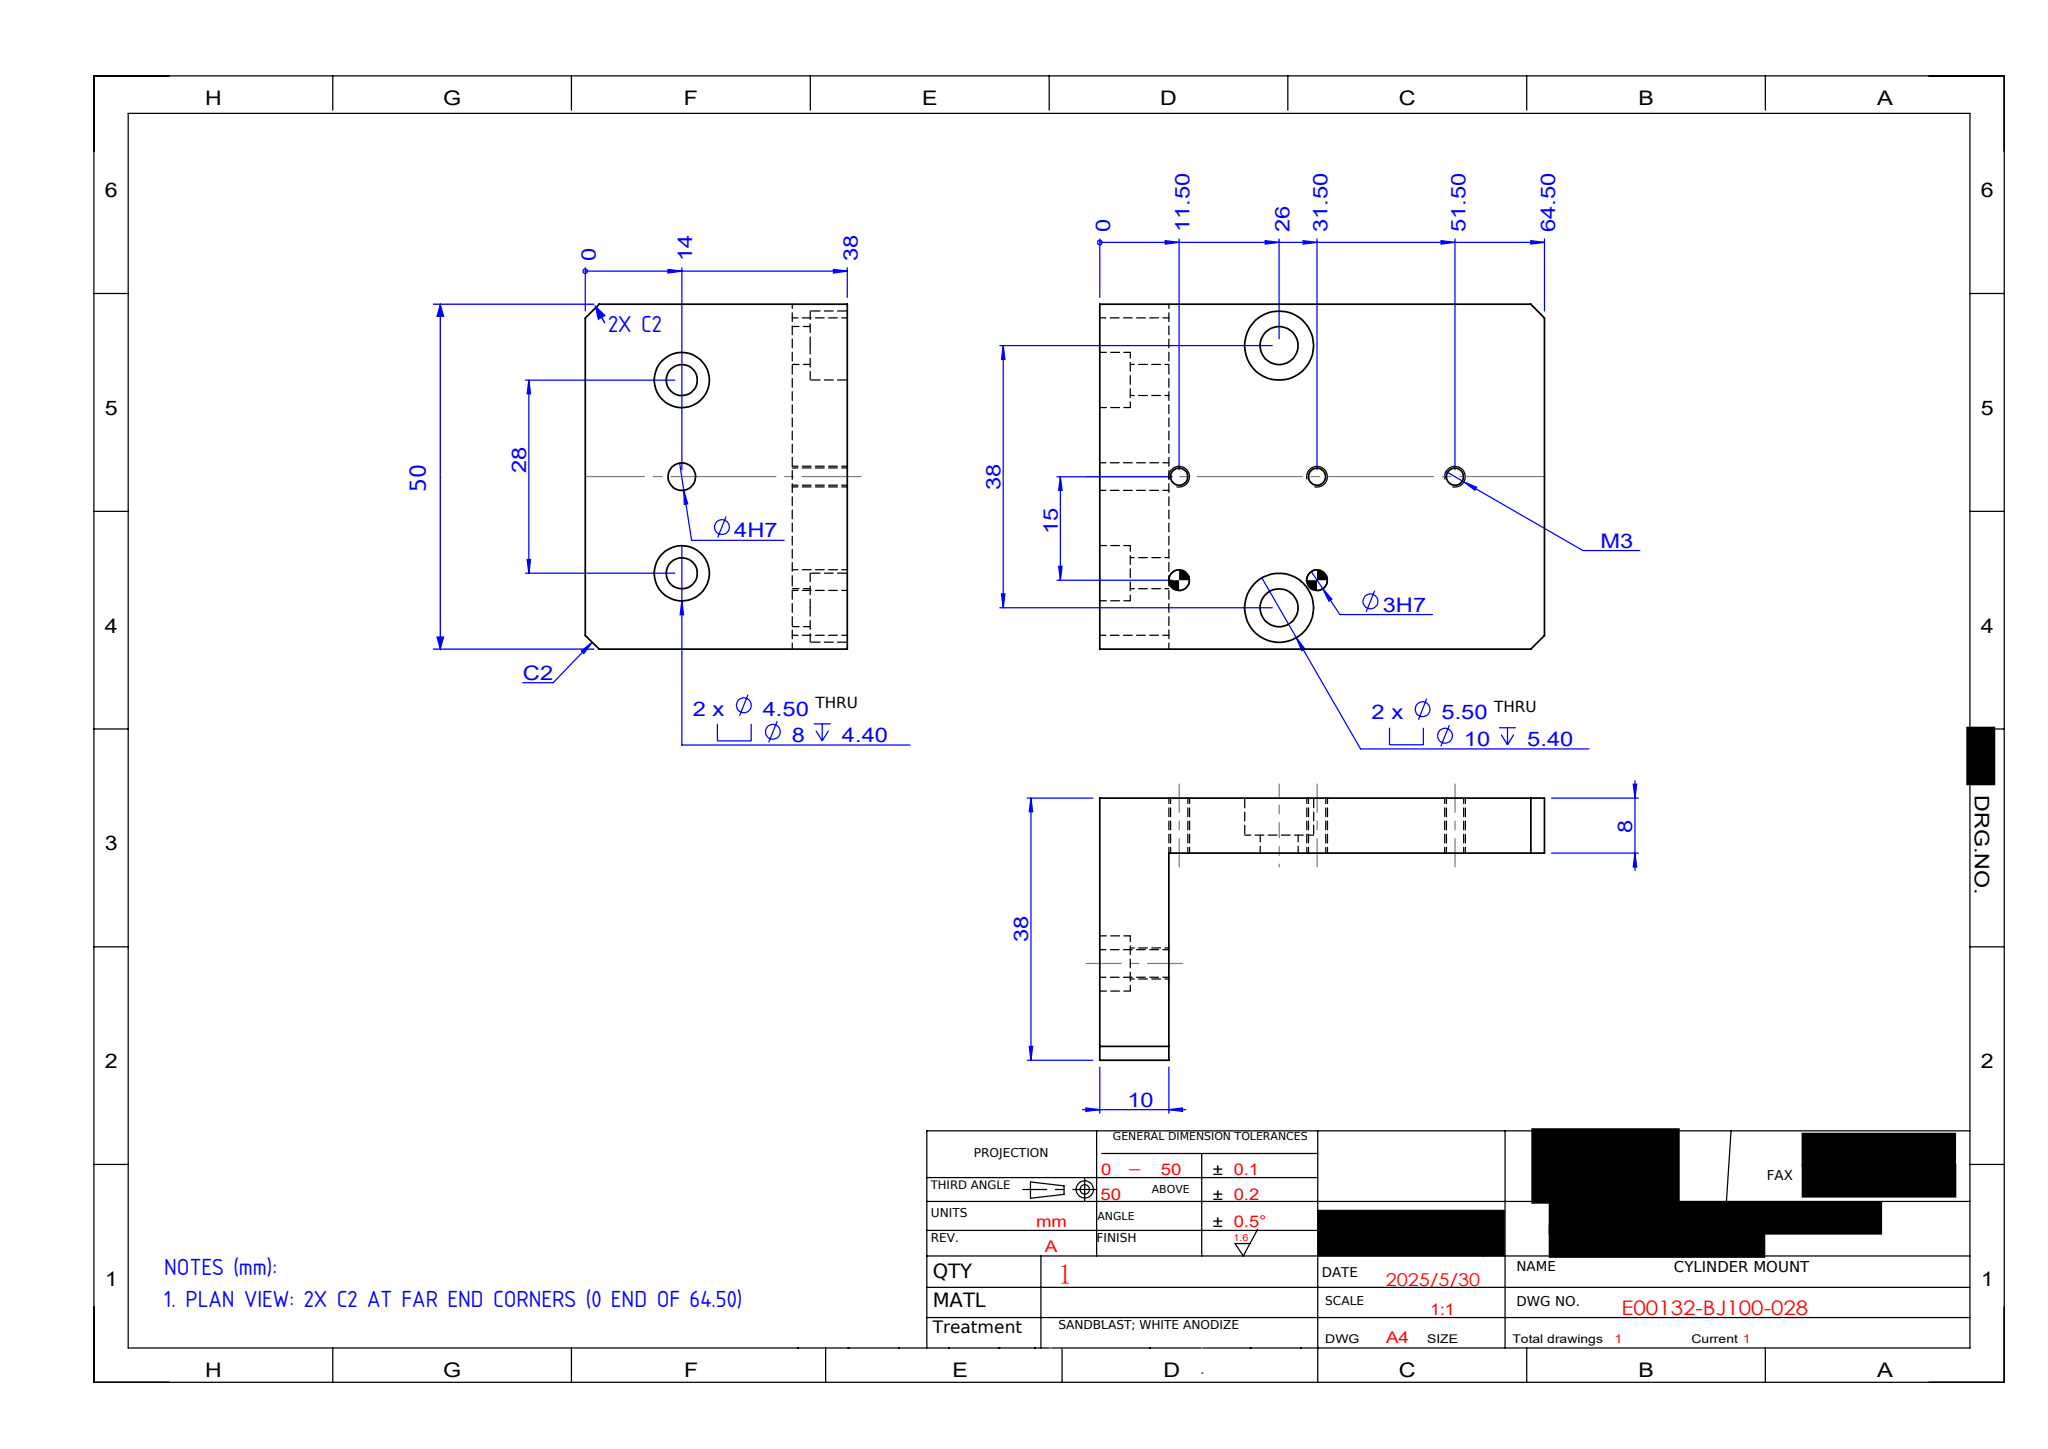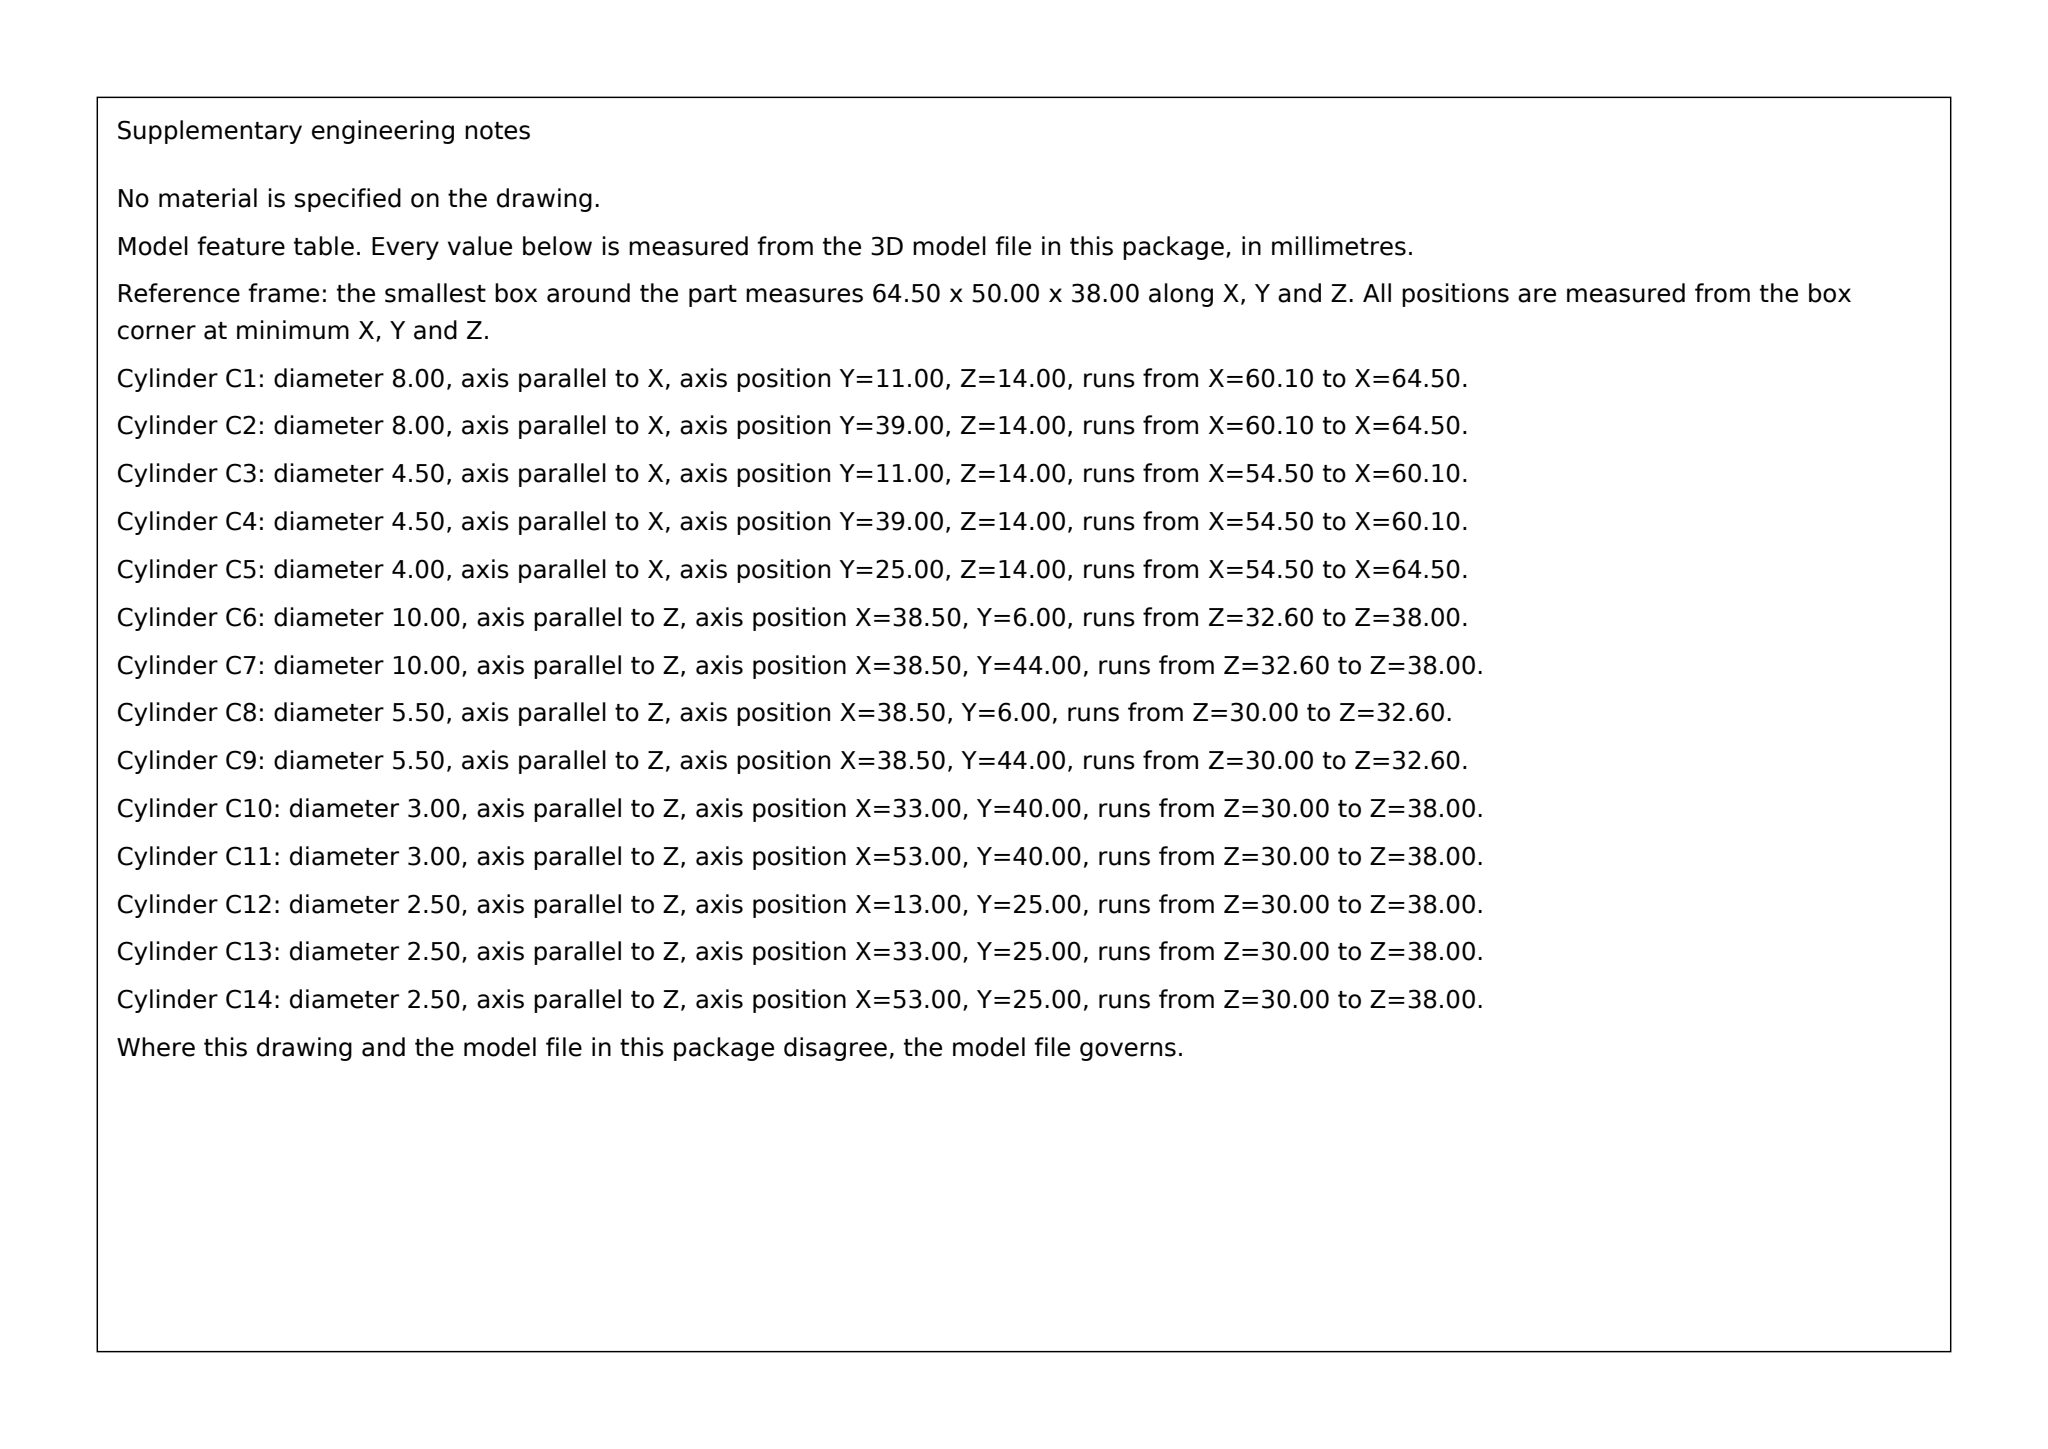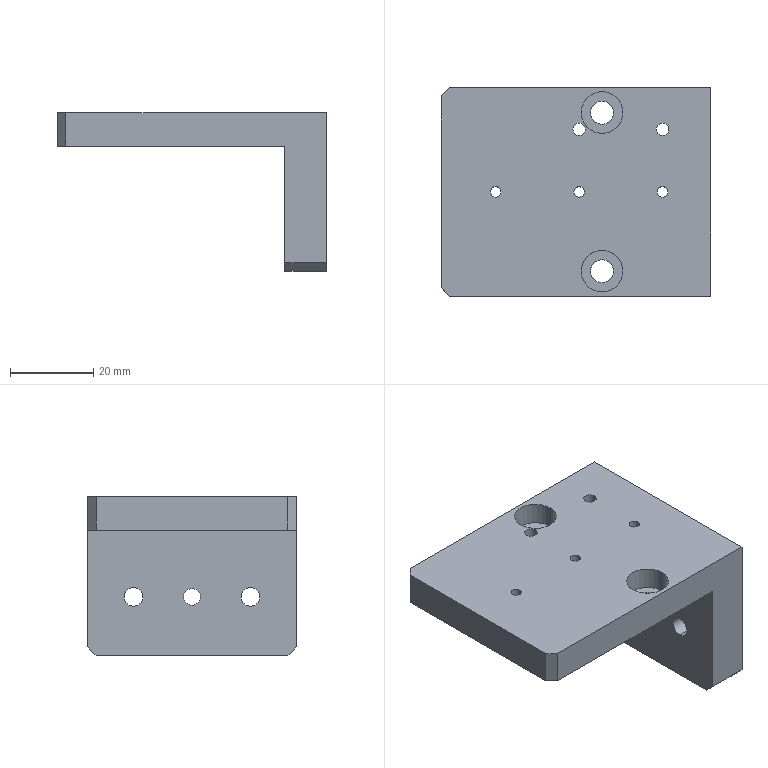Part | SolidWorks | mm | 1 solid | 44 faces | box 64.5 x 50 x 38 mm | volume 38779 mm3 | cylinder 28 | plane 16 | commonest cylinder face diameters 2.5 x6 10 x4 3 x4 8 x4 5.5 x4 4.5 x4 4 x2
Drawing notes:
2X C2 AT LEG FREE-END CORNERS (FRONT VIEW) | from the solid: Leg spans z=0-30 at x=54.5-64.5; two symmetric chamfered corners at z=0 end, y=0 and y=50; size per existing C2 callout
PLAN VIEW: 2X C2 AT FAR END CORNERS (0 END OF 64.50) | from the solid: inclined_planes 45/45/90 at bbox_from [0,0,30] & [0,48,30], size 2x2x8 — two 2x2 chamfers on x=0 end of plate, z 30-38